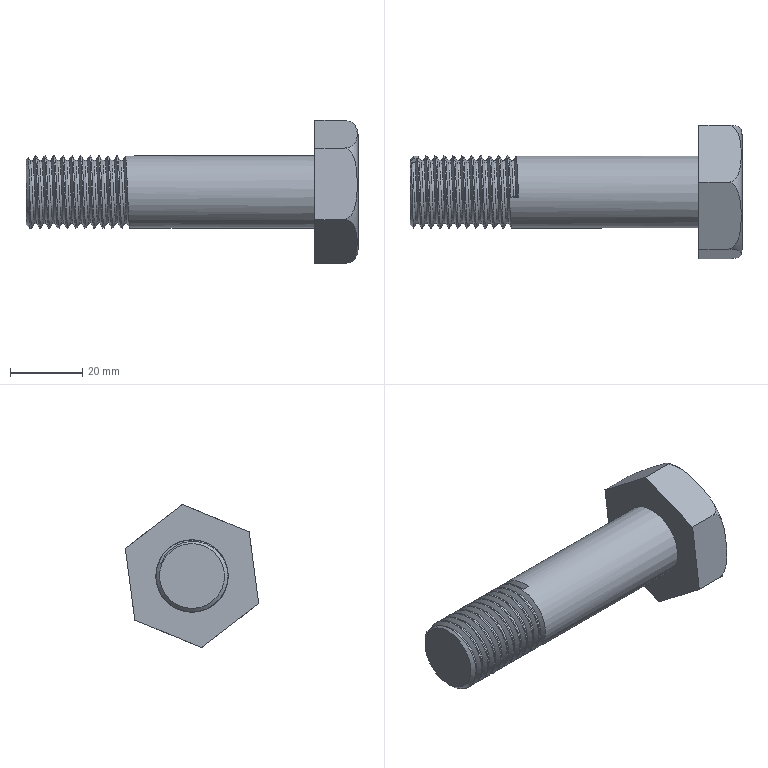Component | NX | CCJ-017_2 | 2 solids | 29 faces | volume 36164 mm3 | cylinder 13 | plane 12 | spline 2 | torus 1 | cone 1 | commonest cylinder face diameters 20 x12 17.5 x1